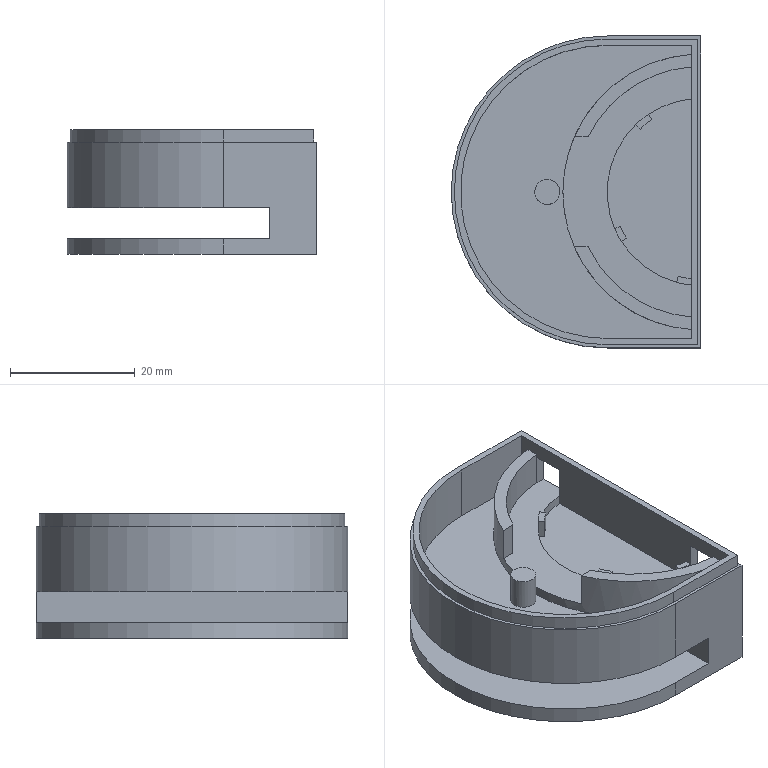Component | NX | HOUSING | 1 solid | 53 faces | volume 15269 mm3 | plane 35 | cylinder 18 | commonest cylinder face diameters 30 x7 28 x3 40.2 x2 50 x2 44.2 x1 47 x1 49 x1 4 x1